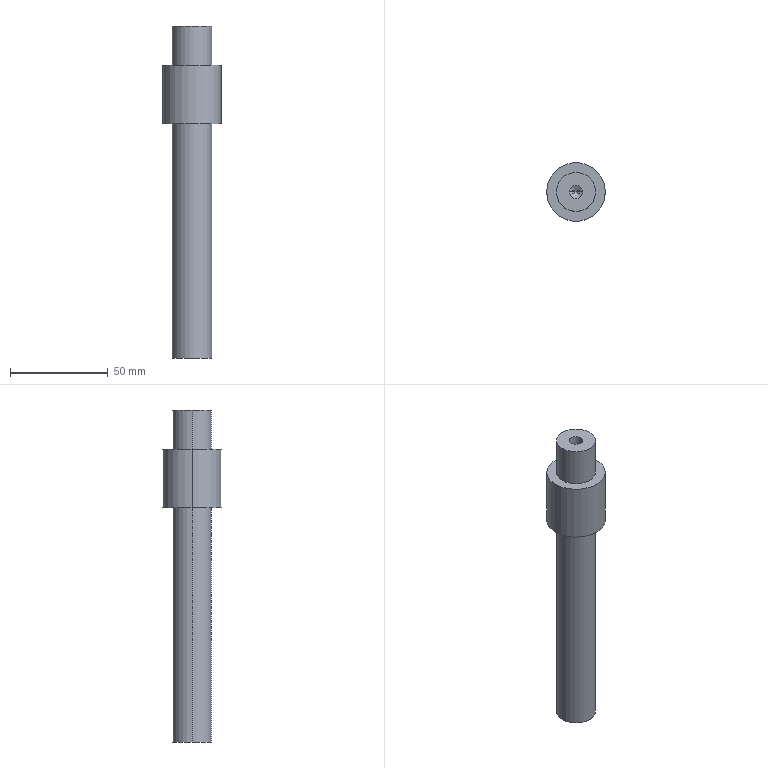Component | SolidWorks | SmallPin-2 | 2 solids | 18 faces | box 30 x 30 x 170 mm | volume 63686 mm3 | cylinder 10 | plane 4 | cone 4 | commonest cylinder face diameters 20 x4 6.8 x4 30 x2
build123d program:
from build123d import *

# Parameters (mm, degrees)
SKETCH1_R                       = 10
BOSS_EXTRUDE2_DEPTH             = 170
M8_TAPPED_HOLE1_D               = 6.8
M8_TAPPED_HOLE1_DEPTH           = 20
M8_TAPPED_HOLE1_TIP             = 2.043
M8_TAPPED_HOLE1_ON_FACE_2_D     = 6.8
M8_TAPPED_HOLE1_ON_FACE_2_DEPTH = 20
M8_TAPPED_HOLE1_ON_FACE_2_TIP   = 2.043
BOSS_EXTRUDE3_START             = -150
SKETCH3_R                       = 15
SKETCH3_R_2                     = 10
BOSS_EXTRUDE3_DEPTH             = 30


with BuildPart() as part:
    # Sketch1 → Boss-Extrude2 (new body)
    with BuildSketch(Plane.XY):
        with Locations((-309.034, -149.403)):
            Circle(SKETCH1_R)
    extrude(amount=-BOSS_EXTRUDE2_DEPTH)

    # M8 Tapped Hole1
    with Locations(Plane(origin=(-309.034, -149.403, 0), x_dir=(1, 0, 0), z_dir=(0, 0, 1))):
        with Locations((0, 0)):
            Hole(M8_TAPPED_HOLE1_D / 2, depth=M8_TAPPED_HOLE1_DEPTH)
            with Locations((0, 0, -(M8_TAPPED_HOLE1_DEPTH + M8_TAPPED_HOLE1_TIP / 2))):  # 118° drill point
                Cone(0, M8_TAPPED_HOLE1_D / 2, M8_TAPPED_HOLE1_TIP, mode=Mode.SUBTRACT)

    # M8 Tapped Hole1 on face 2
    with Locations(Plane(origin=(-309.034, -149.403, -170), x_dir=(-1, 0, 0), z_dir=(0, 0, -1))):
        with Locations((0, 0)):
            Hole(M8_TAPPED_HOLE1_ON_FACE_2_D / 2, depth=M8_TAPPED_HOLE1_ON_FACE_2_DEPTH)
            with Locations((0, 0, -(M8_TAPPED_HOLE1_ON_FACE_2_DEPTH + M8_TAPPED_HOLE1_ON_FACE_2_TIP / 2))):  # 118° drill point
                Cone(0, M8_TAPPED_HOLE1_ON_FACE_2_D / 2, M8_TAPPED_HOLE1_ON_FACE_2_TIP, mode=Mode.SUBTRACT)


with BuildPart() as body_2:
    # Sketch3 → Boss-Extrude3 (new body)
    with BuildSketch(Plane.XY.offset(BOSS_EXTRUDE3_START)):
        with Locations((-309.034, -149.403)):
            Circle(SKETCH3_R)
        with Locations((-309.034, -149.403)):
            Circle(SKETCH3_R_2, mode=Mode.SUBTRACT)
    extrude(amount=BOSS_EXTRUDE3_DEPTH)


solid = Compound([part.part, body_2.part])

# Placed as in the assembly
solid = solid.moved(Location((618.069, -298.805, 0), (180, 0, 0)))
STEP:
#1=COLOUR_RGB('',0.7922,0.8196,0.9333);
#2=FILL_AREA_STYLE_COLOUR('',#1);
#3=FILL_AREA_STYLE('',(#2));
#4=SURFACE_STYLE_FILL_AREA(#3);
#5=SURFACE_SIDE_STYLE('',(#4));
#6=SURFACE_STYLE_USAGE(.BOTH.,#5);
#7=PRESENTATION_STYLE_ASSIGNMENT((#6));
#8=CARTESIAN_POINT('',(12.56,-5.882,4.724));
#9=VERTEX_POINT('',#8);
#10=CARTESIAN_POINT('',(11.773,-5.882,4.724));
#11=VERTEX_POINT('',#10);
#12=CARTESIAN_POINT('',(12.167,-5.882,4.724));
#13=DIRECTION('',(0.,0.,-1.));
#14=DIRECTION('',(-1.,0.,0.));
#15=AXIS2_PLACEMENT_3D('',#12,#13,#14);
#16=CIRCLE('',#15,0.3937);
#17=EDGE_CURVE('',#9,#11,#16,.T.);
#18=ORIENTED_EDGE('',*,*,#17,.T.);
#19=CARTESIAN_POINT('',(11.773,-5.882,5.906));
#20=VERTEX_POINT('',#19);
#21=CARTESIAN_POINT('',(11.773,-5.882,4.724));
#22=DIRECTION('',(0.,0.,1.));
#23=VECTOR('',#22,39.37);
#24=LINE('',#21,#23);
#25=EDGE_CURVE('',#11,#20,#24,.T.);
#26=ORIENTED_EDGE('',*,*,#25,.T.);
#27=CARTESIAN_POINT('',(12.56,-5.882,5.906));
#28=VERTEX_POINT('',#27);
#29=CARTESIAN_POINT('',(12.167,-5.882,5.906));
#30=DIRECTION('',(0.,0.,-1.));
#31=DIRECTION('',(-1.,0.,0.));
#32=AXIS2_PLACEMENT_3D('',#29,#30,#31);
#33=CIRCLE('',#32,0.3937);
#34=EDGE_CURVE('',#28,#20,#33,.T.);
#35=ORIENTED_EDGE('',*,*,#34,.F.);
#36=CARTESIAN_POINT('',(12.56,-5.882,4.724));
#37=DIRECTION('',(0.,0.,1.));
#38=VECTOR('',#37,39.37);
#39=LINE('',#36,#38);
#40=EDGE_CURVE('',#9,#28,#39,.T.);
#41=ORIENTED_EDGE('',*,*,#40,.F.);
#42=EDGE_LOOP('',(#18,#26,#35,#41));
#43=FACE_OUTER_BOUND('',#42,.T.);
#44=CARTESIAN_POINT('',(12.167,-5.882,4.724));
#45=DIRECTION('',(0.,0.,1.));
#46=DIRECTION('',(1.,0.,0.));
#47=AXIS2_PLACEMENT_3D('',#44,#45,#46);
#48=CYLINDRICAL_SURFACE('',#47,0.3937);
#49=ADVANCED_FACE('',(#43),#48,.F.);
#50=CARTESIAN_POINT('',(11.576,-5.882,4.724));
#51=VERTEX_POINT('',#50);
#52=CARTESIAN_POINT('',(12.757,-5.882,4.724));
#53=VERTEX_POINT('',#52);
#54=CARTESIAN_POINT('',(12.167,-5.882,4.724));
#55=DIRECTION('',(0.,0.,-1.));
#56=DIRECTION('',(-1.,0.,0.));
#57=AXIS2_PLACEMENT_3D('',#54,#55,#56);
#58=CIRCLE('',#57,0.5906);
#59=EDGE_CURVE('',#51,#53,#58,.T.);
#60=ORIENTED_EDGE('',*,*,#59,.F.);
#61=CARTESIAN_POINT('',(11.576,-5.882,5.906));
#62=VERTEX_POINT('',#61);
#63=CARTESIAN_POINT('',(11.576,-5.882,4.724));
#64=DIRECTION('',(0.,0.,1.));
#65=VECTOR('',#64,39.37);
#66=LINE('',#63,#65);
#67=EDGE_CURVE('',#51,#62,#66,.T.);
#68=ORIENTED_EDGE('',*,*,#67,.T.);
#69=CARTESIAN_POINT('',(12.757,-5.882,5.906));
#70=VERTEX_POINT('',#69);
#71=CARTESIAN_POINT('',(12.167,-5.882,5.906));
#72=DIRECTION('',(0.,0.,-1.));
#73=DIRECTION('',(-1.,0.,0.));
#74=AXIS2_PLACEMENT_3D('',#71,#72,#73);
#75=CIRCLE('',#74,0.5906);
#76=EDGE_CURVE('',#62,#70,#75,.T.);
#77=ORIENTED_EDGE('',*,*,#76,.T.);
#78=CARTESIAN_POINT('',(12.757,-5.882,4.724));
#79=DIRECTION('',(0.,0.,1.));
#80=VECTOR('',#79,39.37);
#81=LINE('',#78,#80);
#82=EDGE_CURVE('',#53,#70,#81,.T.);
#83=ORIENTED_EDGE('',*,*,#82,.F.);
#84=EDGE_LOOP('',(#60,#68,#77,#83));
#85=FACE_OUTER_BOUND('',#84,.T.);
#86=CARTESIAN_POINT('',(12.167,-5.882,4.724));
#87=DIRECTION('',(0.,0.,1.));
#88=DIRECTION('',(1.,0.,0.));
#89=AXIS2_PLACEMENT_3D('',#86,#87,#88);
#90=CYLINDRICAL_SURFACE('',#89,0.5906);
#91=ADVANCED_FACE('',(#85),#90,.T.);
#92=CARTESIAN_POINT('',(12.167,-5.882,4.724));
#93=DIRECTION('',(0.,0.,-1.));
#94=DIRECTION('',(-1.,0.,0.));
#95=AXIS2_PLACEMENT_3D('',#92,#93,#94);
#96=CIRCLE('',#95,0.5906);
#97=EDGE_CURVE('',#53,#51,#96,.T.);
#98=ORIENTED_EDGE('',*,*,#97,.T.);
#99=ORIENTED_EDGE('',*,*,#59,.T.);
#100=EDGE_LOOP('',(#98,#99));
#101=FACE_OUTER_BOUND('',#100,.T.);
#102=ORIENTED_EDGE('',*,*,#17,.F.);
#103=CARTESIAN_POINT('',(12.167,-5.882,4.724));
#104=DIRECTION('',(0.,0.,-1.));
#105=DIRECTION('',(-1.,0.,0.));
#106=AXIS2_PLACEMENT_3D('',#103,#104,#105);
#107=CIRCLE('',#106,0.3937);
#108=EDGE_CURVE('',#11,#9,#107,.T.);
#109=ORIENTED_EDGE('',*,*,#108,.F.);
#110=EDGE_LOOP('',(#102,#109));
#111=FACE_BOUND('',#110,.T.);
#112=CARTESIAN_POINT('',(12.167,-5.882,4.724));
#113=DIRECTION('',(0.,0.,-1.));
#114=DIRECTION('',(-1.,0.,0.));
#115=AXIS2_PLACEMENT_3D('',#112,#113,#114);
#116=PLANE('',#115);
#117=ADVANCED_FACE('',(#101,#111),#116,.T.);
#118=CARTESIAN_POINT('',(12.167,-5.882,5.906));
#119=DIRECTION('',(0.,0.,-1.));
#120=DIRECTION('',(-1.,0.,0.));
#121=AXIS2_PLACEMENT_3D('',#118,#119,#120);
#122=CIRCLE('',#121,0.5906);
#123=EDGE_CURVE('',#70,#62,#122,.T.);
#124=ORIENTED_EDGE('',*,*,#123,.F.);
#125=ORIENTED_EDGE('',*,*,#76,.F.);
#126=EDGE_LOOP('',(#124,#125));
#127=FACE_OUTER_BOUND('',#126,.T.);
#128=ORIENTED_EDGE('',*,*,#34,.T.);
#129=CARTESIAN_POINT('',(12.167,-5.882,5.906));
#130=DIRECTION('',(0.,0.,-1.));
#131=DIRECTION('',(-1.,0.,0.));
#132=AXIS2_PLACEMENT_3D('',#129,#130,#131);
#133=CIRCLE('',#132,0.3937);
#134=EDGE_CURVE('',#20,#28,#133,.T.);
#135=ORIENTED_EDGE('',*,*,#134,.T.);
#136=EDGE_LOOP('',(#128,#135));
#137=FACE_BOUND('',#136,.T.);
#138=CARTESIAN_POINT('',(12.167,-5.882,5.906));
#139=DIRECTION('',(0.,0.,-1.));
#140=DIRECTION('',(-1.,0.,0.));
#141=AXIS2_PLACEMENT_3D('',#138,#139,#140);
#142=PLANE('',#141);
#143=ADVANCED_FACE('',(#127,#137),#142,.F.);
#144=ORIENTED_EDGE('',*,*,#67,.F.);
#145=ORIENTED_EDGE('',*,*,#97,.F.);
#146=ORIENTED_EDGE('',*,*,#82,.T.);
#147=ORIENTED_EDGE('',*,*,#123,.T.);
#148=EDGE_LOOP('',(#144,#145,#146,#147));
#149=FACE_OUTER_BOUND('',#148,.T.);
#150=CARTESIAN_POINT('',(12.167,-5.882,4.724));
#151=DIRECTION('',(0.,0.,1.));
#152=DIRECTION('',(1.,0.,0.));
#153=AXIS2_PLACEMENT_3D('',#150,#151,#152);
#154=CYLINDRICAL_SURFACE('',#153,0.5906);
#155=ADVANCED_FACE('',(#149),#154,.T.);
#156=ORIENTED_EDGE('',*,*,#25,.F.);
#157=ORIENTED_EDGE('',*,*,#108,.T.);
#158=ORIENTED_EDGE('',*,*,#40,.T.);
#159=ORIENTED_EDGE('',*,*,#134,.F.);
#160=EDGE_LOOP('',(#156,#157,#158,#159));
#161=FACE_OUTER_BOUND('',#160,.T.);
#162=CARTESIAN_POINT('',(12.167,-5.882,4.724));
#163=DIRECTION('',(0.,0.,1.));
#164=DIRECTION('',(1.,0.,0.));
#165=AXIS2_PLACEMENT_3D('',#162,#163,#164);
#166=CYLINDRICAL_SURFACE('',#165,0.3937);
#167=ADVANCED_FACE('',(#161),#166,.F.);
#168=CLOSED_SHELL('',(#49,#91,#117,#143,#155,#167));
#169=MANIFOLD_SOLID_BREP('',#168);
#170=STYLED_ITEM('',(#7),#169);
#171=(LENGTH_UNIT()NAMED_UNIT(*)SI_UNIT($,.METRE.));
#172=LENGTH_MEASURE_WITH_UNIT(LENGTH_MEASURE(0.0254),#171);
#173=DIMENSIONAL_EXPONENTS(1.,0.,0.,0.,0.,0.,0.);
#174=(CONVERSION_BASED_UNIT('',#172)LENGTH_UNIT()NAMED_UNIT(#173));
#175=UNCERTAINTY_MEASURE_WITH_UNIT(LENGTH_MEASURE(0.00001),#174,'','');
#176=(NAMED_UNIT(*)PLANE_ANGLE_UNIT()SI_UNIT($,.RADIAN.));
#177=(NAMED_UNIT(*)SI_UNIT($,.STERADIAN.)SOLID_ANGLE_UNIT());
#178=(GEOMETRIC_REPRESENTATION_CONTEXT(3)GLOBAL_UNCERTAINTY_ASSIGNED_CONTEXT((#175))GLOBAL_UNIT_ASSIGNED_CONTEXT((#174,#176,#177))REPRESENTATION_CONTEXT('',''));
#179=MECHANICAL_DESIGN_GEOMETRIC_PRESENTATION_REPRESENTATION('',(#170),#178);
#180=COLOUR_RGB('',0.7922,0.8196,0.9333);
#181=FILL_AREA_STYLE_COLOUR('',#180);
#182=FILL_AREA_STYLE('',(#181));
#183=SURFACE_STYLE_FILL_AREA(#182);
#184=SURFACE_SIDE_STYLE('',(#183));
#185=SURFACE_STYLE_USAGE(.BOTH.,#184);
#186=PRESENTATION_STYLE_ASSIGNMENT((#185));
#187=CARTESIAN_POINT('',(12.301,-5.882,0.7874));
#188=VERTEX_POINT('',#187);
#189=CARTESIAN_POINT('',(12.033,-5.882,0.7874));
#190=VERTEX_POINT('',#189);
#191=CARTESIAN_POINT('',(12.167,-5.882,0.7874));
#192=DIRECTION('',(0.,0.,-1.));
#193=DIRECTION('',(-1.,0.,0.));
#194=AXIS2_PLACEMENT_3D('',#191,#192,#193);
#195=CIRCLE('',#194,0.1339);
#196=EDGE_CURVE('',#188,#190,#195,.T.);
#197=ORIENTED_EDGE('',*,*,#196,.F.);
#198=CARTESIAN_POINT('',(12.301,-5.882,-0.));
#199=VERTEX_POINT('',#198);
#200=CARTESIAN_POINT('',(12.301,-5.882,0.));
#201=DIRECTION('',(0.,0.,-1.));
#202=VECTOR('',#201,39.37);
#203=LINE('',#200,#202);
#204=EDGE_CURVE('',#188,#199,#203,.T.);
#205=ORIENTED_EDGE('',*,*,#204,.T.);
#206=CARTESIAN_POINT('',(12.033,-5.882,-0.));
#207=VERTEX_POINT('',#206);
#208=CARTESIAN_POINT('',(12.167,-5.882,-0.));
#209=DIRECTION('',(0.,0.,-1.));
#210=DIRECTION('',(-1.,0.,0.));
#211=AXIS2_PLACEMENT_3D('',#208,#209,#210);
#212=CIRCLE('',#211,0.1339);
#213=EDGE_CURVE('',#199,#207,#212,.T.);
#214=ORIENTED_EDGE('',*,*,#213,.T.);
#215=CARTESIAN_POINT('',(12.033,-5.882,0.));
#216=DIRECTION('',(0.,0.,-1.));
#217=VECTOR('',#216,39.37);
#218=LINE('',#215,#217);
#219=EDGE_CURVE('',#190,#207,#218,.T.);
#220=ORIENTED_EDGE('',*,*,#219,.F.);
#221=EDGE_LOOP('',(#197,#205,#214,#220));
#222=FACE_OUTER_BOUND('',#221,.T.);
#223=CARTESIAN_POINT('',(12.167,-5.882,0.));
#224=DIRECTION('',(0.,0.,-1.));
#225=DIRECTION('',(-1.,0.,0.));
#226=AXIS2_PLACEMENT_3D('',#223,#224,#225);
#227=CYLINDRICAL_SURFACE('',#226,0.1339);
#228=ADVANCED_FACE('',(#222),#227,.F.);
#229=CARTESIAN_POINT('',(12.167,-5.882,0.8678));
#230=VERTEX_POINT('',#229);
#231=CARTESIAN_POINT('',(12.033,-5.882,0.7874));
#232=DIRECTION('',(-0.8572,0.,-0.515));
#233=VECTOR('',#232,39.37);
#234=LINE('',#231,#233);
#235=EDGE_CURVE('',#230,#190,#234,.T.);
#236=ORIENTED_EDGE('',*,*,#235,.F.);
#237=CARTESIAN_POINT('',(12.301,-5.882,0.7874));
#238=DIRECTION('',(0.8572,0.,-0.515));
#239=VECTOR('',#238,39.37);
#240=LINE('',#237,#239);
#241=EDGE_CURVE('',#230,#188,#240,.T.);
#242=ORIENTED_EDGE('',*,*,#241,.T.);
#243=ORIENTED_EDGE('',*,*,#196,.T.);
#244=EDGE_LOOP('',(#236,#242,#243));
#245=FACE_OUTER_BOUND('',#244,.T.);
#246=CARTESIAN_POINT('',(12.167,-5.882,0.7874));
#247=DIRECTION('',(0.,0.,-1.));
#248=DIRECTION('',(-1.,0.,0.));
#249=AXIS2_PLACEMENT_3D('',#246,#247,#248);
#250=CONICAL_SURFACE('',#249,0.1339,1.03);
#251=ADVANCED_FACE('',(#245),#250,.F.);
#252=CARTESIAN_POINT('',(12.033,-5.882,5.906));
#253=VERTEX_POINT('',#252);
#254=CARTESIAN_POINT('',(12.301,-5.882,5.906));
#255=VERTEX_POINT('',#254);
#256=CARTESIAN_POINT('',(12.167,-5.882,5.906));
#257=DIRECTION('',(0.,0.,1.));
#258=DIRECTION('',(1.,0.,0.));
#259=AXIS2_PLACEMENT_3D('',#256,#257,#258);
#260=CIRCLE('',#259,0.1339);
#261=EDGE_CURVE('',#253,#255,#260,.T.);
#262=ORIENTED_EDGE('',*,*,#261,.F.);
#263=CARTESIAN_POINT('',(12.033,-5.882,6.693));
#264=VERTEX_POINT('',#263);
#265=CARTESIAN_POINT('',(12.033,-5.882,6.693));
#266=DIRECTION('',(0.,0.,1.));
#267=VECTOR('',#266,39.37);
#268=LINE('',#265,#267);
#269=EDGE_CURVE('',#253,#264,#268,.T.);
#270=ORIENTED_EDGE('',*,*,#269,.T.);
#271=CARTESIAN_POINT('',(12.301,-5.882,6.693));
#272=VERTEX_POINT('',#271);
#273=CARTESIAN_POINT('',(12.167,-5.882,6.693));
#274=DIRECTION('',(0.,0.,1.));
#275=DIRECTION('',(1.,0.,0.));
#276=AXIS2_PLACEMENT_3D('',#273,#274,#275);
#277=CIRCLE('',#276,0.1339);
#278=EDGE_CURVE('',#264,#272,#277,.T.);
#279=ORIENTED_EDGE('',*,*,#278,.T.);
#280=CARTESIAN_POINT('',(12.301,-5.882,6.693));
#281=DIRECTION('',(0.,0.,1.));
#282=VECTOR('',#281,39.37);
#283=LINE('',#280,#282);
#284=EDGE_CURVE('',#255,#272,#283,.T.);
#285=ORIENTED_EDGE('',*,*,#284,.F.);
#286=EDGE_LOOP('',(#262,#270,#279,#285));
#287=FACE_OUTER_BOUND('',#286,.T.);
#288=CARTESIAN_POINT('',(12.167,-5.882,6.693));
#289=DIRECTION('',(0.,0.,1.));
#290=DIRECTION('',(1.,0.,0.));
#291=AXIS2_PLACEMENT_3D('',#288,#289,#290);
#292=CYLINDRICAL_SURFACE('',#291,0.1339);
#293=ADVANCED_FACE('',(#287),#292,.F.);
#294=CARTESIAN_POINT('',(12.167,-5.882,5.825));
#295=VERTEX_POINT('',#294);
#296=CARTESIAN_POINT('',(12.301,-5.882,5.906));
#297=DIRECTION('',(0.8572,0.,0.515));
#298=VECTOR('',#297,39.37);
#299=LINE('',#296,#298);
#300=EDGE_CURVE('',#295,#255,#299,.T.);
#301=ORIENTED_EDGE('',*,*,#300,.F.);
#302=CARTESIAN_POINT('',(12.033,-5.882,5.906));
#303=DIRECTION('',(-0.8572,0.,0.515));
#304=VECTOR('',#303,39.37);
#305=LINE('',#302,#304);
#306=EDGE_CURVE('',#295,#253,#305,.T.);
#307=ORIENTED_EDGE('',*,*,#306,.T.);
#308=ORIENTED_EDGE('',*,*,#261,.T.);
#309=EDGE_LOOP('',(#301,#307,#308));
#310=FACE_OUTER_BOUND('',#309,.T.);
#311=CARTESIAN_POINT('',(12.167,-5.882,5.906));
#312=DIRECTION('',(0.,0.,1.));
#313=DIRECTION('',(1.,0.,0.));
#314=AXIS2_PLACEMENT_3D('',#311,#312,#313);
#315=CONICAL_SURFACE('',#314,0.1339,1.03);
#316=ADVANCED_FACE('',(#310),#315,.F.);
#317=CARTESIAN_POINT('',(11.773,-5.882,6.693));
#318=VERTEX_POINT('',#317);
#319=CARTESIAN_POINT('',(12.56,-5.882,6.693));
#320=VERTEX_POINT('',#319);
#321=CARTESIAN_POINT('',(12.167,-5.882,6.693));
#322=DIRECTION('',(0.,0.,-1.));
#323=DIRECTION('',(-1.,0.,0.));
#324=AXIS2_PLACEMENT_3D('',#321,#322,#323);
#325=CIRCLE('',#324,0.3937);
#326=EDGE_CURVE('',#318,#320,#325,.T.);
#327=ORIENTED_EDGE('',*,*,#326,.T.);
#328=CARTESIAN_POINT('',(12.56,-5.882,0.));
#329=VERTEX_POINT('',#328);
#330=CARTESIAN_POINT('',(12.56,-5.882,6.693));
#331=DIRECTION('',(0.,0.,-1.));
#332=VECTOR('',#331,39.37);
#333=LINE('',#330,#332);
#334=EDGE_CURVE('',#320,#329,#333,.T.);
#335=ORIENTED_EDGE('',*,*,#334,.T.);
#336=CARTESIAN_POINT('',(11.773,-5.882,0.));
#337=VERTEX_POINT('',#336);
#338=CARTESIAN_POINT('',(12.167,-5.882,0.));
#339=DIRECTION('',(0.,0.,-1.));
#340=DIRECTION('',(-1.,0.,0.));
#341=AXIS2_PLACEMENT_3D('',#338,#339,#340);
#342=CIRCLE('',#341,0.3937);
#343=EDGE_CURVE('',#337,#329,#342,.T.);
#344=ORIENTED_EDGE('',*,*,#343,.F.);
#345=CARTESIAN_POINT('',(11.773,-5.882,6.693));
#346=DIRECTION('',(0.,0.,-1.));
#347=VECTOR('',#346,39.37);
#348=LINE('',#345,#347);
#349=EDGE_CURVE('',#318,#337,#348,.T.);
#350=ORIENTED_EDGE('',*,*,#349,.F.);
#351=EDGE_LOOP('',(#327,#335,#344,#350));
#352=FACE_OUTER_BOUND('',#351,.T.);
#353=CARTESIAN_POINT('',(12.167,-5.882,6.693));
#354=DIRECTION('',(0.,0.,-1.));
#355=DIRECTION('',(-1.,0.,0.));
#356=AXIS2_PLACEMENT_3D('',#353,#354,#355);
#357=CYLINDRICAL_SURFACE('',#356,0.3937);
#358=ADVANCED_FACE('',(#352),#357,.T.);
#359=ORIENTED_EDGE('',*,*,#334,.F.);
#360=CARTESIAN_POINT('',(12.167,-5.882,6.693));
#361=DIRECTION('',(0.,0.,-1.));
#362=DIRECTION('',(-1.,0.,0.));
#363=AXIS2_PLACEMENT_3D('',#360,#361,#362);
#364=CIRCLE('',#363,0.3937);
#365=EDGE_CURVE('',#320,#318,#364,.T.);
#366=ORIENTED_EDGE('',*,*,#365,.T.);
#367=ORIENTED_EDGE('',*,*,#349,.T.);
#368=CARTESIAN_POINT('',(12.167,-5.882,0.));
#369=DIRECTION('',(0.,0.,-1.));
#370=DIRECTION('',(-1.,0.,0.));
#371=AXIS2_PLACEMENT_3D('',#368,#369,#370);
#372=CIRCLE('',#371,0.3937);
#373=EDGE_CURVE('',#329,#337,#372,.T.);
#374=ORIENTED_EDGE('',*,*,#373,.F.);
#375=EDGE_LOOP('',(#359,#366,#367,#374));
#376=FACE_OUTER_BOUND('',#375,.T.);
#377=CARTESIAN_POINT('',(12.167,-5.882,6.693));
#378=DIRECTION('',(0.,0.,-1.));
#379=DIRECTION('',(-1.,0.,0.));
#380=AXIS2_PLACEMENT_3D('',#377,#378,#379);
#381=CYLINDRICAL_SURFACE('',#380,0.3937);
#382=ADVANCED_FACE('',(#376),#381,.T.);
#383=CARTESIAN_POINT('',(12.167,-5.882,6.693));
#384=DIRECTION('',(0.,0.,1.));
#385=DIRECTION('',(1.,0.,0.));
#386=AXIS2_PLACEMENT_3D('',#383,#384,#385);
#387=CIRCLE('',#386,0.1339);
#388=EDGE_CURVE('',#272,#264,#387,.T.);
#389=ORIENTED_EDGE('',*,*,#388,.F.);
#390=ORIENTED_EDGE('',*,*,#278,.F.);
#391=EDGE_LOOP('',(#389,#390));
#392=FACE_BOUND('',#391,.T.);
#393=ORIENTED_EDGE('',*,*,#326,.F.);
#394=ORIENTED_EDGE('',*,*,#365,.F.);
#395=EDGE_LOOP('',(#393,#394));
#396=FACE_OUTER_BOUND('',#395,.T.);
#397=CARTESIAN_POINT('',(12.167,-5.882,6.693));
#398=DIRECTION('',(0.,0.,-1.));
#399=DIRECTION('',(-1.,0.,0.));
#400=AXIS2_PLACEMENT_3D('',#397,#398,#399);
#401=PLANE('',#400);
#402=ADVANCED_FACE('',(#392,#396),#401,.F.);
#403=CARTESIAN_POINT('',(12.167,-5.882,-0.));
#404=DIRECTION('',(0.,0.,-1.));
#405=DIRECTION('',(-1.,0.,0.));
#406=AXIS2_PLACEMENT_3D('',#403,#404,#405);
#407=CIRCLE('',#406,0.1339);
#408=EDGE_CURVE('',#207,#199,#407,.T.);
#409=ORIENTED_EDGE('',*,*,#408,.F.);
#410=ORIENTED_EDGE('',*,*,#213,.F.);
#411=EDGE_LOOP('',(#409,#410));
#412=FACE_BOUND('',#411,.T.);
#413=ORIENTED_EDGE('',*,*,#343,.T.);
#414=ORIENTED_EDGE('',*,*,#373,.T.);
#415=EDGE_LOOP('',(#413,#414));
#416=FACE_OUTER_BOUND('',#415,.T.);
#417=CARTESIAN_POINT('',(12.167,-5.882,0.));
#418=DIRECTION('',(0.,0.,-1.));
#419=DIRECTION('',(-1.,0.,0.));
#420=AXIS2_PLACEMENT_3D('',#417,#418,#419);
#421=PLANE('',#420);
#422=ADVANCED_FACE('',(#412,#416),#421,.T.);
#423=ORIENTED_EDGE('',*,*,#306,.F.);
#424=ORIENTED_EDGE('',*,*,#300,.T.);
#425=CARTESIAN_POINT('',(12.167,-5.882,5.906));
#426=DIRECTION('',(0.,0.,1.));
#427=DIRECTION('',(1.,0.,0.));
#428=AXIS2_PLACEMENT_3D('',#425,#426,#427);
#429=CIRCLE('',#428,0.1339);
#430=EDGE_CURVE('',#255,#253,#429,.T.);
#431=ORIENTED_EDGE('',*,*,#430,.T.);
#432=EDGE_LOOP('',(#423,#424,#431));
#433=FACE_OUTER_BOUND('',#432,.T.);
#434=CARTESIAN_POINT('',(12.167,-5.882,5.906));
#435=DIRECTION('',(0.,0.,1.));
#436=DIRECTION('',(1.,0.,0.));
#437=AXIS2_PLACEMENT_3D('',#434,#435,#436);
#438=CONICAL_SURFACE('',#437,0.1339,1.03);
#439=ADVANCED_FACE('',(#433),#438,.F.);
#440=ORIENTED_EDGE('',*,*,#269,.F.);
#441=ORIENTED_EDGE('',*,*,#430,.F.);
#442=ORIENTED_EDGE('',*,*,#284,.T.);
#443=ORIENTED_EDGE('',*,*,#388,.T.);
#444=EDGE_LOOP('',(#440,#441,#442,#443));
#445=FACE_OUTER_BOUND('',#444,.T.);
#446=CARTESIAN_POINT('',(12.167,-5.882,6.693));
#447=DIRECTION('',(0.,0.,1.));
#448=DIRECTION('',(1.,0.,0.));
#449=AXIS2_PLACEMENT_3D('',#446,#447,#448);
#450=CYLINDRICAL_SURFACE('',#449,0.1339);
#451=ADVANCED_FACE('',(#445),#450,.F.);
#452=ORIENTED_EDGE('',*,*,#241,.F.);
#453=ORIENTED_EDGE('',*,*,#235,.T.);
#454=CARTESIAN_POINT('',(12.167,-5.882,0.7874));
#455=DIRECTION('',(0.,0.,-1.));
#456=DIRECTION('',(-1.,0.,0.));
#457=AXIS2_PLACEMENT_3D('',#454,#455,#456);
#458=CIRCLE('',#457,0.1339);
#459=EDGE_CURVE('',#190,#188,#458,.T.);
#460=ORIENTED_EDGE('',*,*,#459,.T.);
#461=EDGE_LOOP('',(#452,#453,#460));
#462=FACE_OUTER_BOUND('',#461,.T.);
#463=CARTESIAN_POINT('',(12.167,-5.882,0.7874));
#464=DIRECTION('',(0.,0.,-1.));
#465=DIRECTION('',(-1.,0.,0.));
#466=AXIS2_PLACEMENT_3D('',#463,#464,#465);
#467=CONICAL_SURFACE('',#466,0.1339,1.03);
#468=ADVANCED_FACE('',(#462),#467,.F.);
#469=ORIENTED_EDGE('',*,*,#204,.F.);
#470=ORIENTED_EDGE('',*,*,#459,.F.);
#471=ORIENTED_EDGE('',*,*,#219,.T.);
#472=ORIENTED_EDGE('',*,*,#408,.T.);
#473=EDGE_LOOP('',(#469,#470,#471,#472));
#474=FACE_OUTER_BOUND('',#473,.T.);
#475=CARTESIAN_POINT('',(12.167,-5.882,0.));
#476=DIRECTION('',(0.,0.,-1.));
#477=DIRECTION('',(-1.,0.,0.));
#478=AXIS2_PLACEMENT_3D('',#475,#476,#477);
#479=CYLINDRICAL_SURFACE('',#478,0.1339);
#480=ADVANCED_FACE('',(#474),#479,.F.);
#481=CLOSED_SHELL('',(#228,#251,#293,#316,#358,#382,#402,#422,#439,#451,#468,#480));
#482=MANIFOLD_SOLID_BREP('',#481);
#483=STYLED_ITEM('',(#186),#482);
#484=PRESENTATION_LAYER_ASSIGNMENT('','',(#483));
#485=CARTESIAN_POINT('',(0.,0.,0.));
#486=DIRECTION('',(0.,0.,1.));
#487=DIRECTION('',(1.,0.,0.));
#488=AXIS2_PLACEMENT_3D('',#485,#486,#487);
#489=(LENGTH_UNIT()NAMED_UNIT(*)SI_UNIT($,.METRE.));
#490=LENGTH_MEASURE_WITH_UNIT(LENGTH_MEASURE(0.0254),#489);
#491=DIMENSIONAL_EXPONENTS(1.,0.,0.,0.,0.,0.,0.);
#492=(CONVERSION_BASED_UNIT('',#490)LENGTH_UNIT()NAMED_UNIT(#491));
#493=UNCERTAINTY_MEASURE_WITH_UNIT(LENGTH_MEASURE(0.00001),#492,'','');
#494=(NAMED_UNIT(*)PLANE_ANGLE_UNIT()SI_UNIT($,.RADIAN.));
#495=(NAMED_UNIT(*)SI_UNIT($,.STERADIAN.)SOLID_ANGLE_UNIT());
#496=(GEOMETRIC_REPRESENTATION_CONTEXT(3)GLOBAL_UNCERTAINTY_ASSIGNED_CONTEXT((#493))GLOBAL_UNIT_ASSIGNED_CONTEXT((#492,#494,#495))REPRESENTATION_CONTEXT('',''));
#497=ADVANCED_BREP_SHAPE_REPRESENTATION('',(#169,#482,#488),#496);
#498=PRESENTATION_LAYER_ASSIGNMENT('','',(#170));
#499=(LENGTH_UNIT()NAMED_UNIT(*)SI_UNIT($,.METRE.));
#500=LENGTH_MEASURE_WITH_UNIT(LENGTH_MEASURE(0.0254),#499);
#501=DIMENSIONAL_EXPONENTS(1.,0.,0.,0.,0.,0.,0.);
#502=(CONVERSION_BASED_UNIT('',#500)LENGTH_UNIT()NAMED_UNIT(#501));
#503=UNCERTAINTY_MEASURE_WITH_UNIT(LENGTH_MEASURE(0.00001),#502,'','');
#504=(NAMED_UNIT(*)PLANE_ANGLE_UNIT()SI_UNIT($,.RADIAN.));
#505=(NAMED_UNIT(*)SI_UNIT($,.STERADIAN.)SOLID_ANGLE_UNIT());
#506=(GEOMETRIC_REPRESENTATION_CONTEXT(3)GLOBAL_UNCERTAINTY_ASSIGNED_CONTEXT((#503))GLOBAL_UNIT_ASSIGNED_CONTEXT((#502,#504,#505))REPRESENTATION_CONTEXT('',''));
#507=MECHANICAL_DESIGN_GEOMETRIC_PRESENTATION_REPRESENTATION('',(#483),#506);